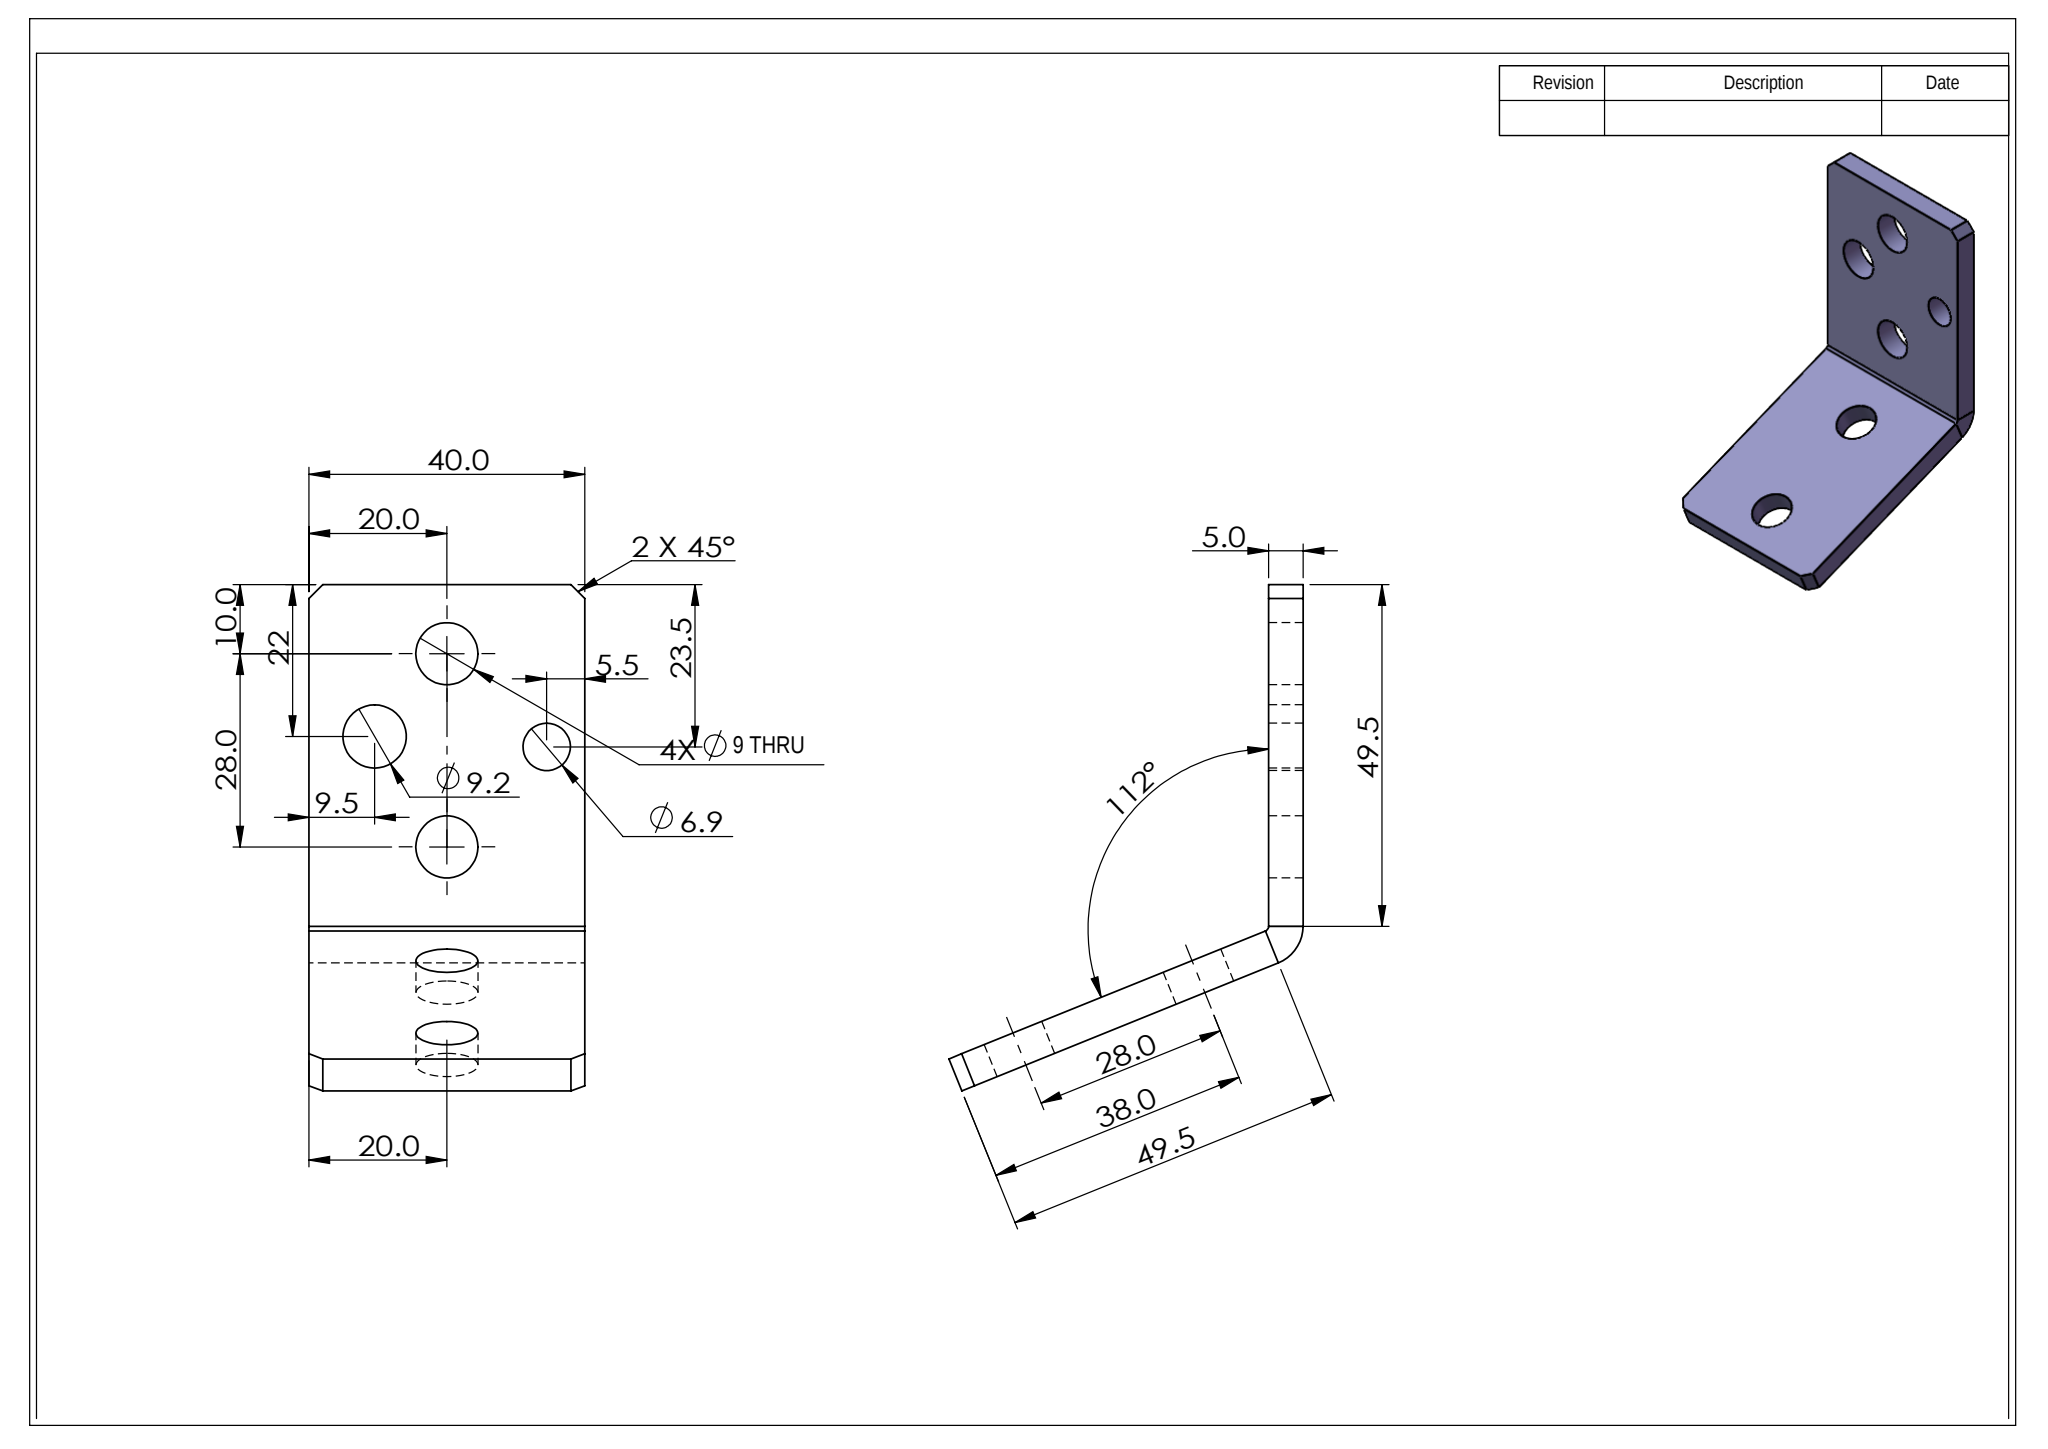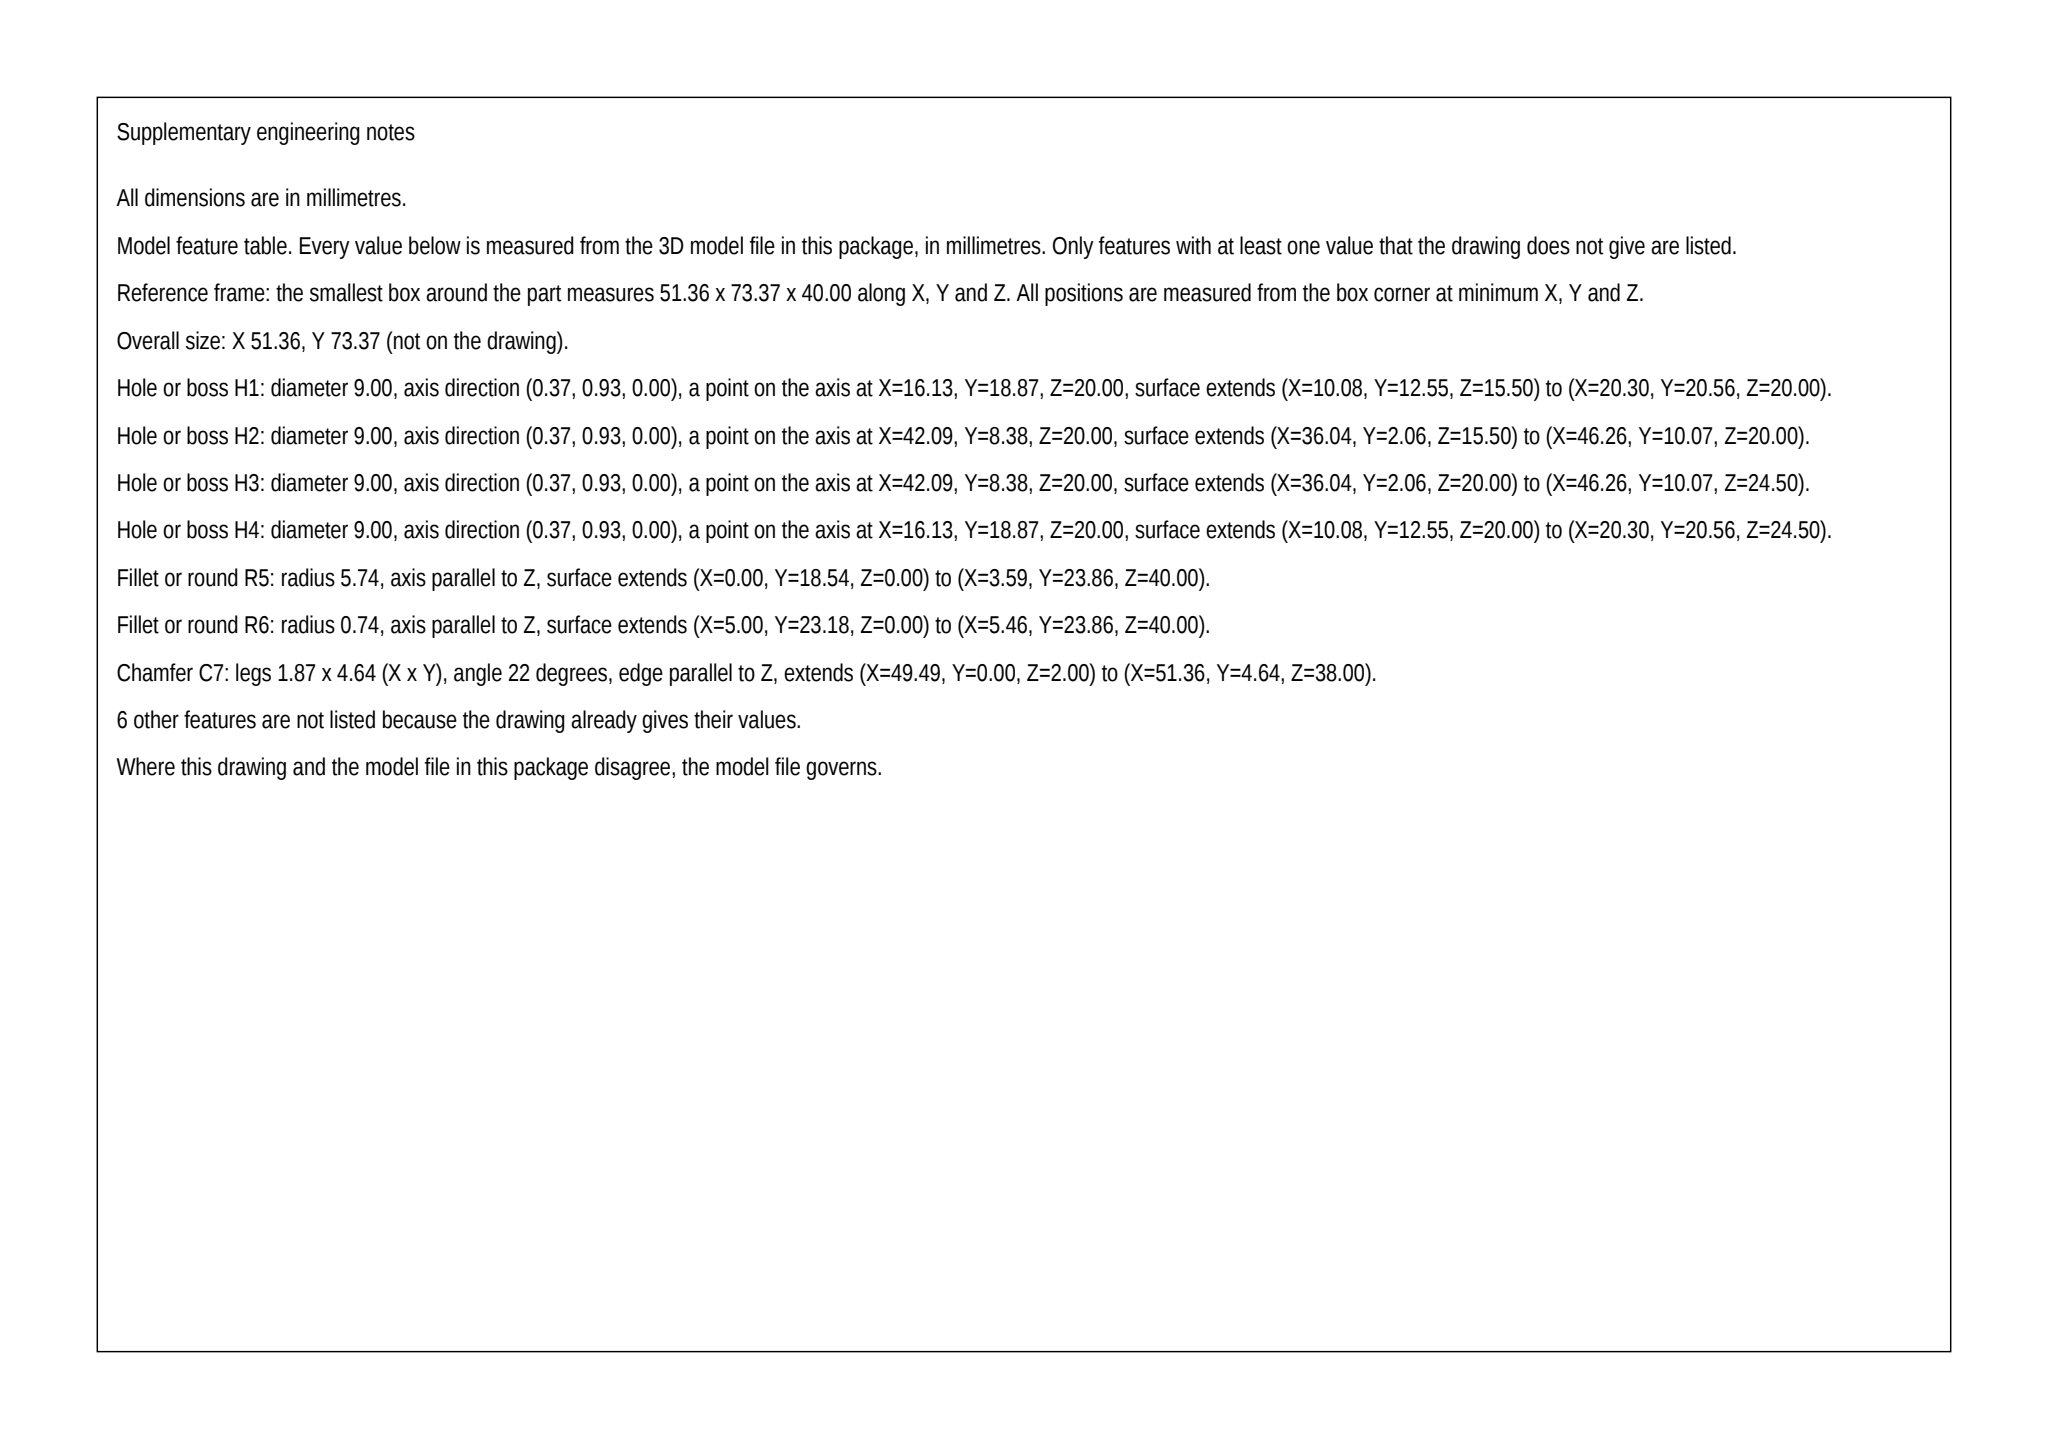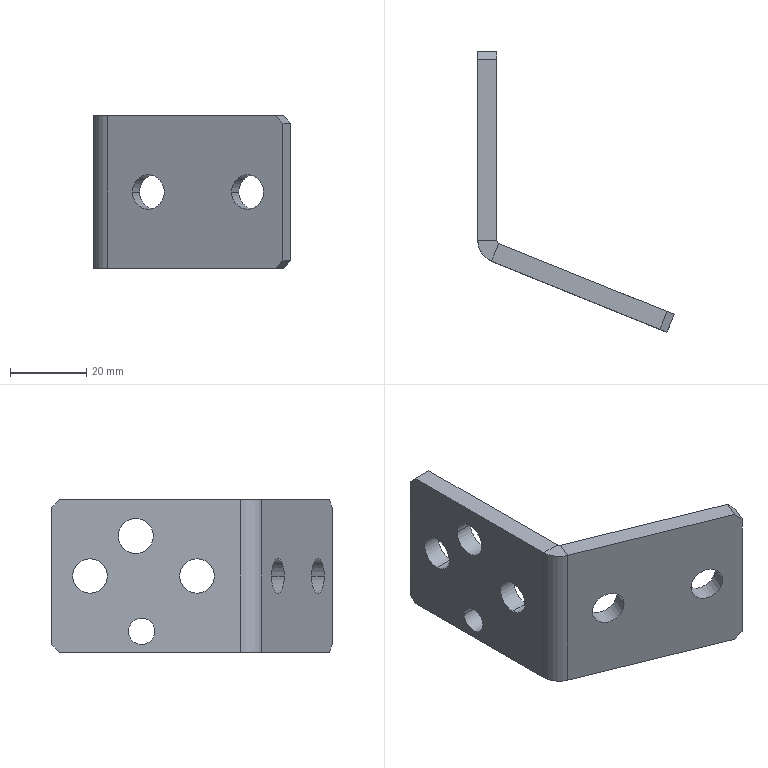Part | SolidWorks | mm | 1 solid | 30 faces | box 51.36 x 73.37 x 40 mm | volume 18742 mm3 | plane 16 | cylinder 14 | commonest cylinder face diameters 9 x8 9.172 x2 6.867 x2 1.473 x1 11.473 x1